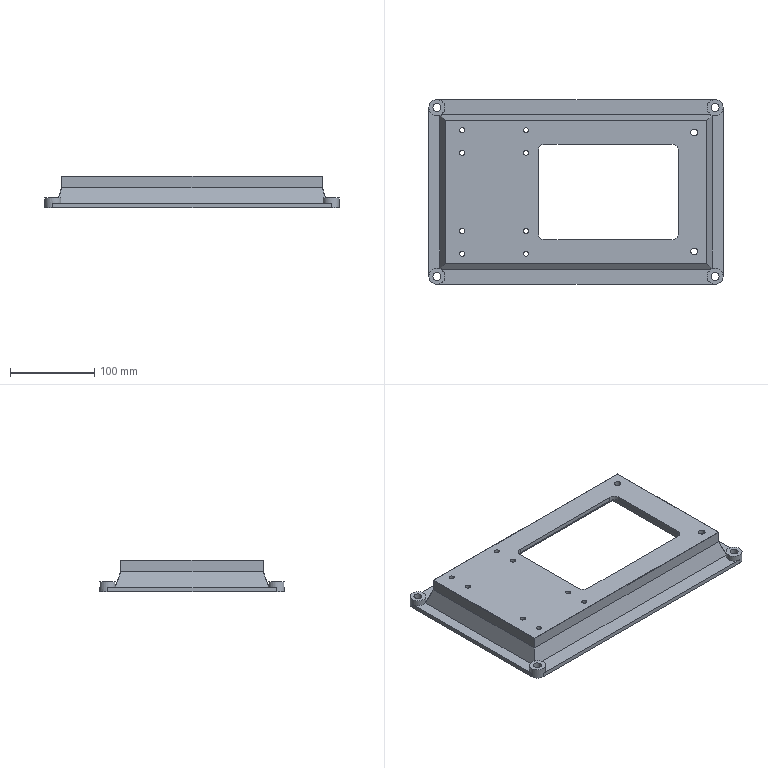Component | NX | BASE | 1 solid | 71 faces | volume 453588 mm3 | plane 49 | cylinder 22 | commonest cylinder face diameters 6 x8 19 x4 9.5 x4 16 x4 8 x2